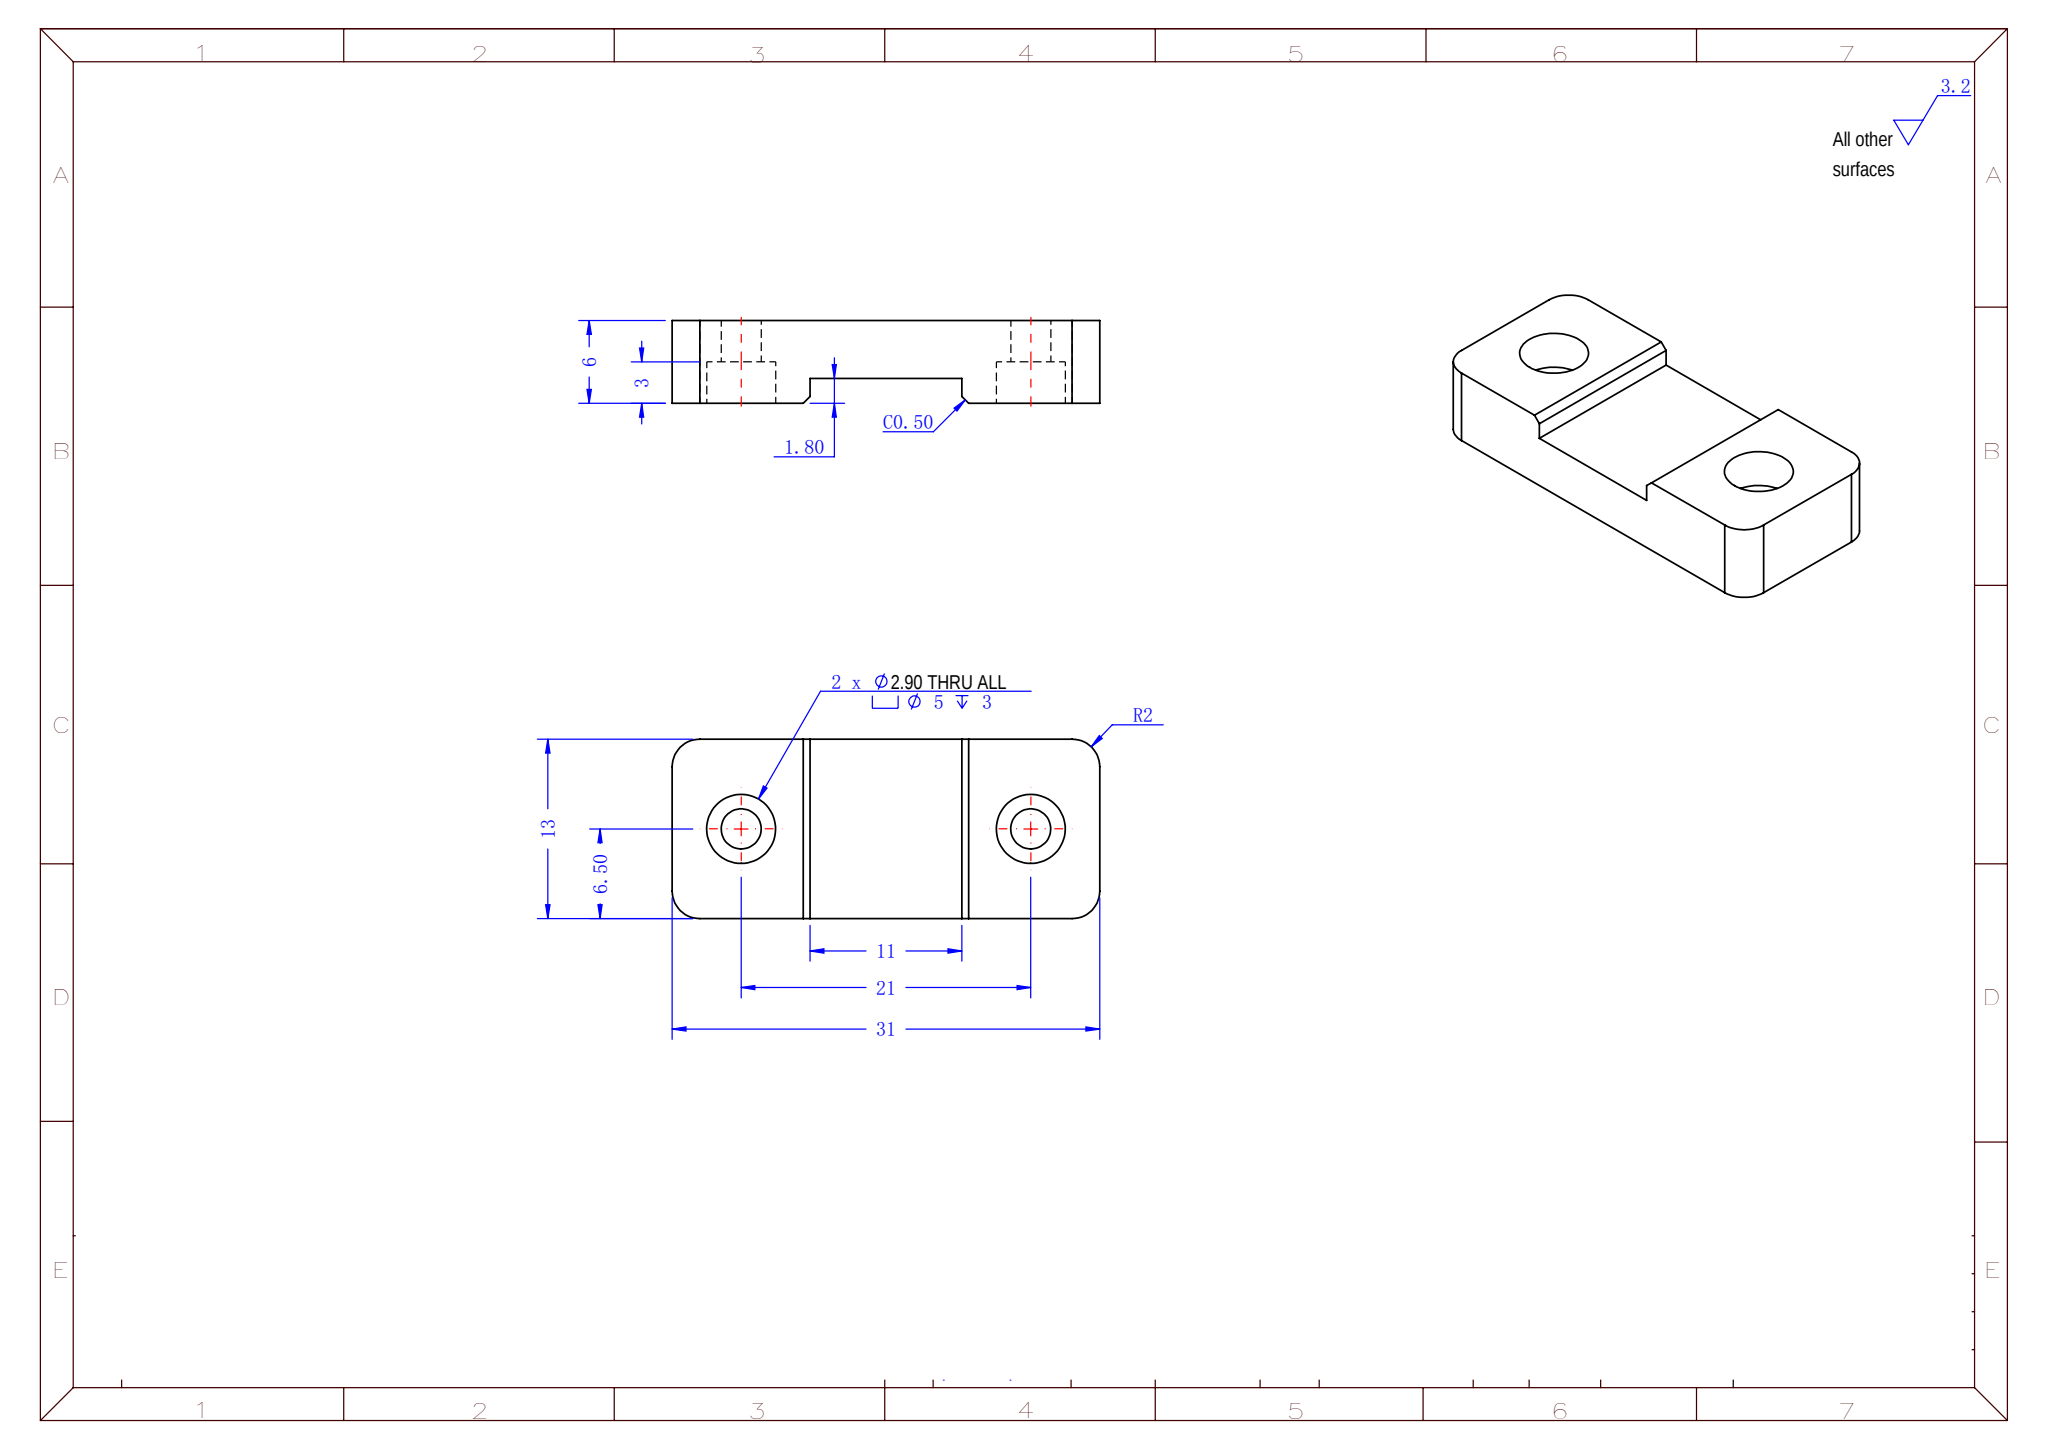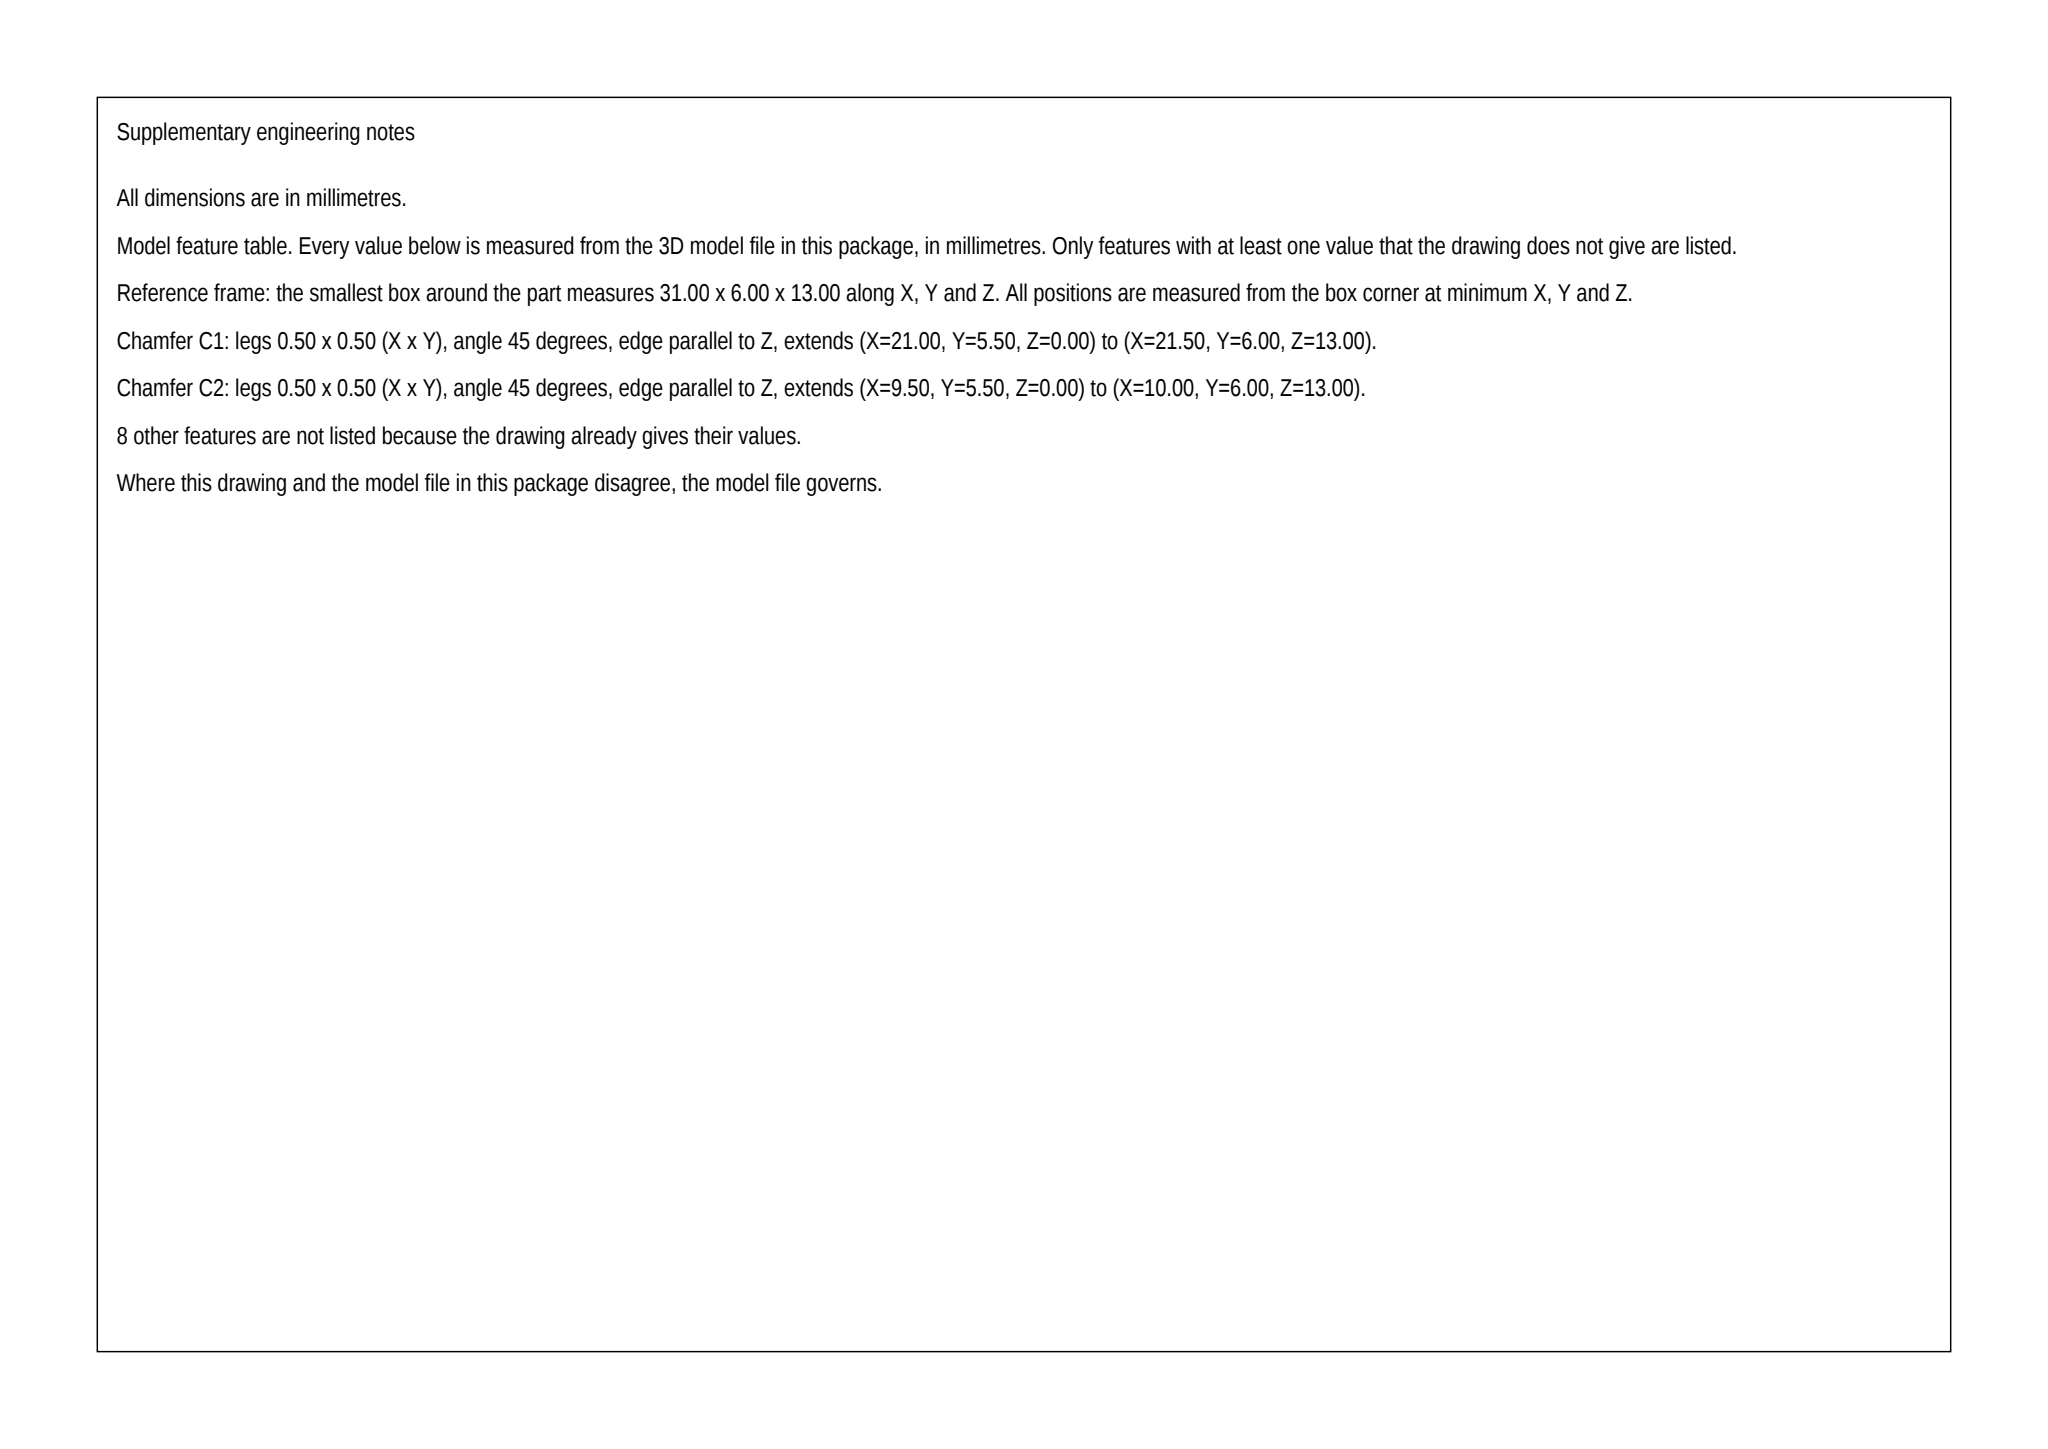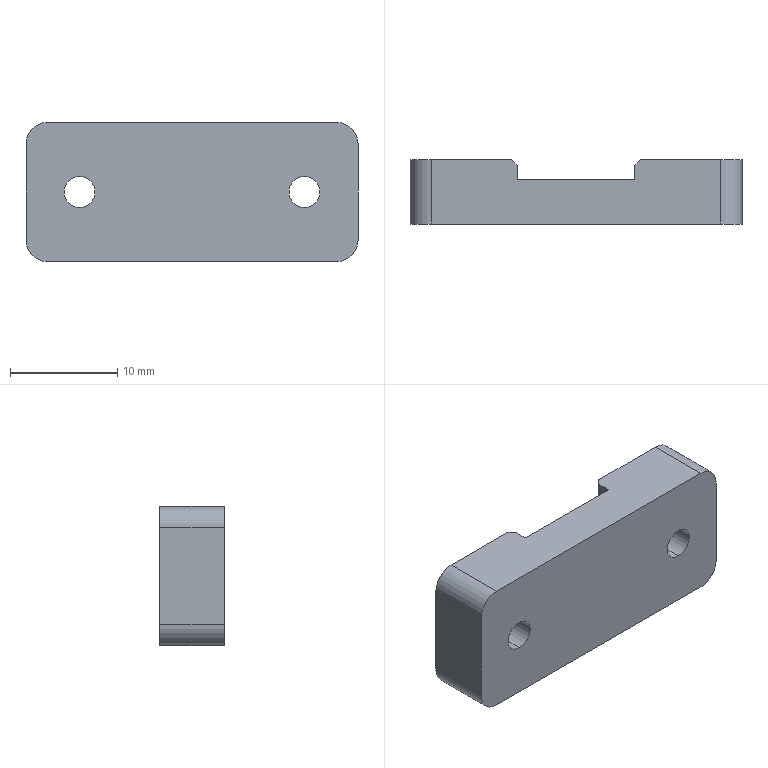Part | SolidWorks | mm | 1 solid | 26 faces | box 31 x 6 x 13 mm | volume 1979 mm3 | plane 14 | cylinder 12 | commonest cylinder face diameters 5 x4 2.9 x4 4 x4
build123d program:
from build123d import *

# Parameters (mm, degrees)
SKETCH1_W                                            = 31
SKETCH1_H                                            = 13
BOSS_EXTRUDE1_DEPTH                                  = 3
FILLET1_R                                            = 2
SKETCH3_W                                            = 11
SKETCH3_H                                            = 1.8
CUT_EXTRUDE2_DEPTH                                   = 21.451
CYLINDRICAL_COUNTERSUNK_HOLE_FOR_M2_5_HE_D           = 2.9
CYLINDRICAL_COUNTERSUNK_HOLE_FOR_M2_5_HE_CBORE_D     = 5
CYLINDRICAL_COUNTERSUNK_HOLE_FOR_M2_5_HE_CBORE_DEPTH = 3
CHAMFER1_SIZE                                        = 0.5


with BuildPart() as part:
    # Sketch1 → Boss-Extrude1 (new, symmetric)
    with BuildSketch(Plane(origin=(0, 0, 0), x_dir=(1, 0, 0), z_dir=(0, 1, 0))):
        Rectangle(SKETCH1_W, SKETCH1_H)
    extrude(amount=BOSS_EXTRUDE1_DEPTH, both=True)

    # Fillet1
    fillet1_edges = [part.edges().sort_by_distance(p)[0] for p in [
        (15.5, 0, 6.5),
        (-15.5, 0, 6.5),
        (-15.5, 0, -6.5),
        (15.5, 0, -6.5),
    ]]
    fillet(fillet1_edges, radius=FILLET1_R)

    # Sketch3 → Cut-Extrude2 (cut, through all)
    with BuildSketch(Plane(origin=(0, 0, -6.5), x_dir=(-1, 0, 0), z_dir=(0, 0, -1))):
        with Locations((0, 2.1)):
            Rectangle(SKETCH3_W, SKETCH3_H)
    extrude(amount=-CUT_EXTRUDE2_DEPTH, mode=Mode.SUBTRACT)

    # Cylindrical Countersunk Hole for M2.5 He (through all)
    with Locations(Plane(origin=(0, 3, 0), x_dir=(1, 0, 0), z_dir=(0, 1, 0))):
        with Locations((10.5, 0), (-10.5, 0)):
            CounterBoreHole(CYLINDRICAL_COUNTERSUNK_HOLE_FOR_M2_5_HE_D / 2, CYLINDRICAL_COUNTERSUNK_HOLE_FOR_M2_5_HE_CBORE_D / 2, CYLINDRICAL_COUNTERSUNK_HOLE_FOR_M2_5_HE_CBORE_DEPTH)

    # Chamfer1
    chamfer1_edges = [part.edges().sort_by_distance(p)[0] for p in [
        (5.5, 3, 0),
        (-5.5, 3, 0),
    ]]
    chamfer(chamfer1_edges, length=CHAMFER1_SIZE)


solid = part.part
STEP:
#1=CARTESIAN_POINT('',(10.5,0.,-2.5));
#2=VERTEX_POINT('',#1);
#3=CARTESIAN_POINT('',(10.5,0.,2.5));
#4=VERTEX_POINT('',#3);
#5=CARTESIAN_POINT('',(10.5,0.,0.));
#6=DIRECTION('',(0.,1.,0.));
#7=DIRECTION('',(0.,0.,1.));
#8=AXIS2_PLACEMENT_3D('',#5,#6,#7);
#9=CIRCLE('',#8,2.5);
#10=EDGE_CURVE('',#2,#4,#9,.T.);
#11=ORIENTED_EDGE('',*,*,#10,.F.);
#12=CARTESIAN_POINT('',(10.5,3.,-2.5));
#13=VERTEX_POINT('',#12);
#14=CARTESIAN_POINT('',(10.5,3.,-2.5));
#15=DIRECTION('',(0.,1.,0.));
#16=VECTOR('',#15,1000.);
#17=LINE('',#14,#16);
#18=EDGE_CURVE('',#2,#13,#17,.T.);
#19=ORIENTED_EDGE('',*,*,#18,.T.);
#20=CARTESIAN_POINT('',(10.5,3.,2.5));
#21=VERTEX_POINT('',#20);
#22=CARTESIAN_POINT('',(10.5,3.,0.));
#23=DIRECTION('',(0.,1.,0.));
#24=DIRECTION('',(0.,0.,1.));
#25=AXIS2_PLACEMENT_3D('',#22,#23,#24);
#26=CIRCLE('',#25,2.5);
#27=EDGE_CURVE('',#13,#21,#26,.T.);
#28=ORIENTED_EDGE('',*,*,#27,.T.);
#29=CARTESIAN_POINT('',(10.5,3.,2.5));
#30=DIRECTION('',(0.,1.,0.));
#31=VECTOR('',#30,1000.);
#32=LINE('',#29,#31);
#33=EDGE_CURVE('',#4,#21,#32,.T.);
#34=ORIENTED_EDGE('',*,*,#33,.F.);
#35=EDGE_LOOP('',(#11,#19,#28,#34));
#36=FACE_OUTER_BOUND('',#35,.T.);
#37=CARTESIAN_POINT('',(10.5,3.,0.));
#38=DIRECTION('',(0.,1.,0.));
#39=DIRECTION('',(0.,0.,1.));
#40=AXIS2_PLACEMENT_3D('',#37,#38,#39);
#41=CYLINDRICAL_SURFACE('',#40,2.5);
#42=ADVANCED_FACE('',(#36),#41,.F.);
#43=CARTESIAN_POINT('',(10.5,-3.,-1.45));
#44=VERTEX_POINT('',#43);
#45=CARTESIAN_POINT('',(10.5,-3.,1.45));
#46=VERTEX_POINT('',#45);
#47=CARTESIAN_POINT('',(10.5,-3.,0.));
#48=DIRECTION('',(0.,1.,0.));
#49=DIRECTION('',(0.,0.,1.));
#50=AXIS2_PLACEMENT_3D('',#47,#48,#49);
#51=CIRCLE('',#50,1.45);
#52=EDGE_CURVE('',#44,#46,#51,.T.);
#53=ORIENTED_EDGE('',*,*,#52,.F.);
#54=CARTESIAN_POINT('',(10.5,0.,-1.45));
#55=VERTEX_POINT('',#54);
#56=CARTESIAN_POINT('',(10.5,3.,-1.45));
#57=DIRECTION('',(0.,1.,0.));
#58=VECTOR('',#57,1000.);
#59=LINE('',#56,#58);
#60=EDGE_CURVE('',#44,#55,#59,.T.);
#61=ORIENTED_EDGE('',*,*,#60,.T.);
#62=CARTESIAN_POINT('',(10.5,0.,1.45));
#63=VERTEX_POINT('',#62);
#64=CARTESIAN_POINT('',(10.5,0.,0.));
#65=DIRECTION('',(0.,1.,0.));
#66=DIRECTION('',(0.,0.,1.));
#67=AXIS2_PLACEMENT_3D('',#64,#65,#66);
#68=CIRCLE('',#67,1.45);
#69=EDGE_CURVE('',#55,#63,#68,.T.);
#70=ORIENTED_EDGE('',*,*,#69,.T.);
#71=CARTESIAN_POINT('',(10.5,3.,1.45));
#72=DIRECTION('',(0.,1.,0.));
#73=VECTOR('',#72,1000.);
#74=LINE('',#71,#73);
#75=EDGE_CURVE('',#46,#63,#74,.T.);
#76=ORIENTED_EDGE('',*,*,#75,.F.);
#77=EDGE_LOOP('',(#53,#61,#70,#76));
#78=FACE_OUTER_BOUND('',#77,.T.);
#79=CARTESIAN_POINT('',(10.5,3.,0.));
#80=DIRECTION('',(0.,1.,0.));
#81=DIRECTION('',(0.,0.,1.));
#82=AXIS2_PLACEMENT_3D('',#79,#80,#81);
#83=CYLINDRICAL_SURFACE('',#82,1.45);
#84=ADVANCED_FACE('',(#78),#83,.F.);
#85=CARTESIAN_POINT('',(-10.5,0.,-2.5));
#86=VERTEX_POINT('',#85);
#87=CARTESIAN_POINT('',(-10.5,0.,2.5));
#88=VERTEX_POINT('',#87);
#89=CARTESIAN_POINT('',(-10.5,0.,0.));
#90=DIRECTION('',(0.,1.,0.));
#91=DIRECTION('',(0.,0.,1.));
#92=AXIS2_PLACEMENT_3D('',#89,#90,#91);
#93=CIRCLE('',#92,2.5);
#94=EDGE_CURVE('',#86,#88,#93,.T.);
#95=ORIENTED_EDGE('',*,*,#94,.F.);
#96=CARTESIAN_POINT('',(-10.5,3.,-2.5));
#97=VERTEX_POINT('',#96);
#98=CARTESIAN_POINT('',(-10.5,3.,-2.5));
#99=DIRECTION('',(0.,1.,0.));
#100=VECTOR('',#99,1000.);
#101=LINE('',#98,#100);
#102=EDGE_CURVE('',#86,#97,#101,.T.);
#103=ORIENTED_EDGE('',*,*,#102,.T.);
#104=CARTESIAN_POINT('',(-10.5,3.,2.5));
#105=VERTEX_POINT('',#104);
#106=CARTESIAN_POINT('',(-10.5,3.,0.));
#107=DIRECTION('',(0.,1.,0.));
#108=DIRECTION('',(0.,0.,1.));
#109=AXIS2_PLACEMENT_3D('',#106,#107,#108);
#110=CIRCLE('',#109,2.5);
#111=EDGE_CURVE('',#97,#105,#110,.T.);
#112=ORIENTED_EDGE('',*,*,#111,.T.);
#113=CARTESIAN_POINT('',(-10.5,3.,2.5));
#114=DIRECTION('',(0.,1.,0.));
#115=VECTOR('',#114,1000.);
#116=LINE('',#113,#115);
#117=EDGE_CURVE('',#88,#105,#116,.T.);
#118=ORIENTED_EDGE('',*,*,#117,.F.);
#119=EDGE_LOOP('',(#95,#103,#112,#118));
#120=FACE_OUTER_BOUND('',#119,.T.);
#121=CARTESIAN_POINT('',(-10.5,3.,0.));
#122=DIRECTION('',(0.,1.,0.));
#123=DIRECTION('',(0.,0.,1.));
#124=AXIS2_PLACEMENT_3D('',#121,#122,#123);
#125=CYLINDRICAL_SURFACE('',#124,2.5);
#126=ADVANCED_FACE('',(#120),#125,.F.);
#127=CARTESIAN_POINT('',(-10.5,-3.,-1.45));
#128=VERTEX_POINT('',#127);
#129=CARTESIAN_POINT('',(-10.5,-3.,1.45));
#130=VERTEX_POINT('',#129);
#131=CARTESIAN_POINT('',(-10.5,-3.,0.));
#132=DIRECTION('',(0.,1.,0.));
#133=DIRECTION('',(0.,0.,1.));
#134=AXIS2_PLACEMENT_3D('',#131,#132,#133);
#135=CIRCLE('',#134,1.45);
#136=EDGE_CURVE('',#128,#130,#135,.T.);
#137=ORIENTED_EDGE('',*,*,#136,.F.);
#138=CARTESIAN_POINT('',(-10.5,0.,-1.45));
#139=VERTEX_POINT('',#138);
#140=CARTESIAN_POINT('',(-10.5,3.,-1.45));
#141=DIRECTION('',(0.,1.,0.));
#142=VECTOR('',#141,1000.);
#143=LINE('',#140,#142);
#144=EDGE_CURVE('',#128,#139,#143,.T.);
#145=ORIENTED_EDGE('',*,*,#144,.T.);
#146=CARTESIAN_POINT('',(-10.5,0.,1.45));
#147=VERTEX_POINT('',#146);
#148=CARTESIAN_POINT('',(-10.5,0.,0.));
#149=DIRECTION('',(0.,1.,0.));
#150=DIRECTION('',(0.,0.,1.));
#151=AXIS2_PLACEMENT_3D('',#148,#149,#150);
#152=CIRCLE('',#151,1.45);
#153=EDGE_CURVE('',#139,#147,#152,.T.);
#154=ORIENTED_EDGE('',*,*,#153,.T.);
#155=CARTESIAN_POINT('',(-10.5,3.,1.45));
#156=DIRECTION('',(0.,1.,0.));
#157=VECTOR('',#156,1000.);
#158=LINE('',#155,#157);
#159=EDGE_CURVE('',#130,#147,#158,.T.);
#160=ORIENTED_EDGE('',*,*,#159,.F.);
#161=EDGE_LOOP('',(#137,#145,#154,#160));
#162=FACE_OUTER_BOUND('',#161,.T.);
#163=CARTESIAN_POINT('',(-10.5,3.,0.));
#164=DIRECTION('',(0.,1.,0.));
#165=DIRECTION('',(0.,0.,1.));
#166=AXIS2_PLACEMENT_3D('',#163,#164,#165);
#167=CYLINDRICAL_SURFACE('',#166,1.45);
#168=ADVANCED_FACE('',(#162),#167,.F.);
#169=CARTESIAN_POINT('',(-10.5,3.,0.));
#170=DIRECTION('',(0.,1.,0.));
#171=DIRECTION('',(0.,0.,1.));
#172=AXIS2_PLACEMENT_3D('',#169,#170,#171);
#173=CIRCLE('',#172,2.5);
#174=EDGE_CURVE('',#105,#97,#173,.T.);
#175=ORIENTED_EDGE('',*,*,#174,.F.);
#176=ORIENTED_EDGE('',*,*,#111,.F.);
#177=EDGE_LOOP('',(#175,#176));
#178=FACE_BOUND('',#177,.T.);
#179=CARTESIAN_POINT('',(-13.5,3.,6.5));
#180=VERTEX_POINT('',#179);
#181=CARTESIAN_POINT('',(-6.,3.,6.5));
#182=VERTEX_POINT('',#181);
#183=CARTESIAN_POINT('',(-15.5,3.,6.5));
#184=DIRECTION('',(1.,0.,0.));
#185=VECTOR('',#184,1000.);
#186=LINE('',#183,#185);
#187=EDGE_CURVE('',#180,#182,#186,.T.);
#188=ORIENTED_EDGE('',*,*,#187,.T.);
#189=CARTESIAN_POINT('',(-6.,3.,-6.5));
#190=VERTEX_POINT('',#189);
#191=CARTESIAN_POINT('',(-6.,3.,-6.5));
#192=DIRECTION('',(0.,0.,-1.));
#193=VECTOR('',#192,1000.);
#194=LINE('',#191,#193);
#195=EDGE_CURVE('',#182,#190,#194,.T.);
#196=ORIENTED_EDGE('',*,*,#195,.T.);
#197=CARTESIAN_POINT('',(-13.5,3.,-6.5));
#198=VERTEX_POINT('',#197);
#199=CARTESIAN_POINT('',(-15.5,3.,-6.5));
#200=DIRECTION('',(-1.,0.,0.));
#201=VECTOR('',#200,1000.);
#202=LINE('',#199,#201);
#203=EDGE_CURVE('',#190,#198,#202,.T.);
#204=ORIENTED_EDGE('',*,*,#203,.T.);
#205=CARTESIAN_POINT('',(-15.5,3.,-4.5));
#206=VERTEX_POINT('',#205);
#207=CARTESIAN_POINT('',(-13.5,3.,-4.5));
#208=DIRECTION('',(0.,1.,0.));
#209=DIRECTION('',(0.,0.,1.));
#210=AXIS2_PLACEMENT_3D('',#207,#208,#209);
#211=CIRCLE('',#210,2.);
#212=EDGE_CURVE('',#198,#206,#211,.T.);
#213=ORIENTED_EDGE('',*,*,#212,.T.);
#214=CARTESIAN_POINT('',(-15.5,3.,4.5));
#215=VERTEX_POINT('',#214);
#216=CARTESIAN_POINT('',(-15.5,3.,-6.5));
#217=DIRECTION('',(0.,0.,1.));
#218=VECTOR('',#217,1000.);
#219=LINE('',#216,#218);
#220=EDGE_CURVE('',#206,#215,#219,.T.);
#221=ORIENTED_EDGE('',*,*,#220,.T.);
#222=CARTESIAN_POINT('',(-13.5,3.,4.5));
#223=DIRECTION('',(0.,1.,0.));
#224=DIRECTION('',(0.,0.,1.));
#225=AXIS2_PLACEMENT_3D('',#222,#223,#224);
#226=CIRCLE('',#225,2.);
#227=EDGE_CURVE('',#215,#180,#226,.T.);
#228=ORIENTED_EDGE('',*,*,#227,.T.);
#229=EDGE_LOOP('',(#188,#196,#204,#213,#221,#228));
#230=FACE_OUTER_BOUND('',#229,.T.);
#231=CARTESIAN_POINT('',(0.,3.,0.));
#232=DIRECTION('',(0.,1.,0.));
#233=DIRECTION('',(0.,0.,1.));
#234=AXIS2_PLACEMENT_3D('',#231,#232,#233);
#235=PLANE('',#234);
#236=ADVANCED_FACE('',(#178,#230),#235,.T.);
#237=CARTESIAN_POINT('',(15.5,3.,4.5));
#238=VERTEX_POINT('',#237);
#239=CARTESIAN_POINT('',(15.5,3.,-4.5));
#240=VERTEX_POINT('',#239);
#241=CARTESIAN_POINT('',(15.5,3.,-6.5));
#242=DIRECTION('',(-0.,0.,-1.));
#243=VECTOR('',#242,1000.);
#244=LINE('',#241,#243);
#245=EDGE_CURVE('',#238,#240,#244,.T.);
#246=ORIENTED_EDGE('',*,*,#245,.F.);
#247=CARTESIAN_POINT('',(15.5,-3.,4.5));
#248=VERTEX_POINT('',#247);
#249=CARTESIAN_POINT('',(15.5,3.,4.5));
#250=DIRECTION('',(0.,-1.,0.));
#251=VECTOR('',#250,1000.);
#252=LINE('',#249,#251);
#253=EDGE_CURVE('',#238,#248,#252,.T.);
#254=ORIENTED_EDGE('',*,*,#253,.T.);
#255=CARTESIAN_POINT('',(15.5,-3.,-4.5));
#256=VERTEX_POINT('',#255);
#257=CARTESIAN_POINT('',(15.5,-3.,-6.5));
#258=DIRECTION('',(-0.,0.,-1.));
#259=VECTOR('',#258,1000.);
#260=LINE('',#257,#259);
#261=EDGE_CURVE('',#248,#256,#260,.T.);
#262=ORIENTED_EDGE('',*,*,#261,.T.);
#263=CARTESIAN_POINT('',(15.5,3.,-4.5));
#264=DIRECTION('',(0.,1.,0.));
#265=VECTOR('',#264,1000.);
#266=LINE('',#263,#265);
#267=EDGE_CURVE('',#256,#240,#266,.T.);
#268=ORIENTED_EDGE('',*,*,#267,.T.);
#269=EDGE_LOOP('',(#246,#254,#262,#268));
#270=FACE_OUTER_BOUND('',#269,.T.);
#271=CARTESIAN_POINT('',(15.5,3.,-6.5));
#272=DIRECTION('',(-1.,0.,0.));
#273=DIRECTION('',(0.,0.,1.));
#274=AXIS2_PLACEMENT_3D('',#271,#272,#273);
#275=PLANE('',#274);
#276=ADVANCED_FACE('',(#270),#275,.F.);
#277=CARTESIAN_POINT('',(5.5,2.5,-6.5));
#278=VERTEX_POINT('',#277);
#279=CARTESIAN_POINT('',(5.5,1.2,-6.5));
#280=VERTEX_POINT('',#279);
#281=CARTESIAN_POINT('',(5.5,3.,-6.5));
#282=DIRECTION('',(0.,-1.,0.));
#283=VECTOR('',#282,1000.);
#284=LINE('',#281,#283);
#285=EDGE_CURVE('',#278,#280,#284,.T.);
#286=ORIENTED_EDGE('',*,*,#285,.F.);
#287=CARTESIAN_POINT('',(6.,3.,-6.5));
#288=VERTEX_POINT('',#287);
#289=CARTESIAN_POINT('',(5.5,2.5,-6.5));
#290=DIRECTION('',(0.7071,0.7071,0.));
#291=VECTOR('',#290,1000.);
#292=LINE('',#289,#291);
#293=EDGE_CURVE('',#278,#288,#292,.T.);
#294=ORIENTED_EDGE('',*,*,#293,.T.);
#295=CARTESIAN_POINT('',(13.5,3.,-6.5));
#296=VERTEX_POINT('',#295);
#297=CARTESIAN_POINT('',(-15.5,3.,-6.5));
#298=DIRECTION('',(-1.,0.,0.));
#299=VECTOR('',#298,1000.);
#300=LINE('',#297,#299);
#301=EDGE_CURVE('',#296,#288,#300,.T.);
#302=ORIENTED_EDGE('',*,*,#301,.F.);
#303=CARTESIAN_POINT('',(13.5,-3.,-6.5));
#304=VERTEX_POINT('',#303);
#305=CARTESIAN_POINT('',(13.5,3.,-6.5));
#306=DIRECTION('',(0.,-1.,0.));
#307=VECTOR('',#306,1000.);
#308=LINE('',#305,#307);
#309=EDGE_CURVE('',#296,#304,#308,.T.);
#310=ORIENTED_EDGE('',*,*,#309,.T.);
#311=CARTESIAN_POINT('',(-13.5,-3.,-6.5));
#312=VERTEX_POINT('',#311);
#313=CARTESIAN_POINT('',(-15.5,-3.,-6.5));
#314=DIRECTION('',(-1.,0.,0.));
#315=VECTOR('',#314,1000.);
#316=LINE('',#313,#315);
#317=EDGE_CURVE('',#304,#312,#316,.T.);
#318=ORIENTED_EDGE('',*,*,#317,.T.);
#319=CARTESIAN_POINT('',(-13.5,3.,-6.5));
#320=DIRECTION('',(0.,1.,0.));
#321=VECTOR('',#320,1000.);
#322=LINE('',#319,#321);
#323=EDGE_CURVE('',#312,#198,#322,.T.);
#324=ORIENTED_EDGE('',*,*,#323,.T.);
#325=ORIENTED_EDGE('',*,*,#203,.F.);
#326=CARTESIAN_POINT('',(-5.5,2.5,-6.5));
#327=VERTEX_POINT('',#326);
#328=CARTESIAN_POINT('',(-6.,3.,-6.5));
#329=DIRECTION('',(0.7071,-0.7071,0.));
#330=VECTOR('',#329,1000.);
#331=LINE('',#328,#330);
#332=EDGE_CURVE('',#190,#327,#331,.T.);
#333=ORIENTED_EDGE('',*,*,#332,.T.);
#334=CARTESIAN_POINT('',(-5.5,1.2,-6.5));
#335=VERTEX_POINT('',#334);
#336=CARTESIAN_POINT('',(-5.5,1.2,-6.5));
#337=DIRECTION('',(0.,1.,0.));
#338=VECTOR('',#337,1000.);
#339=LINE('',#336,#338);
#340=EDGE_CURVE('',#335,#327,#339,.T.);
#341=ORIENTED_EDGE('',*,*,#340,.F.);
#342=CARTESIAN_POINT('',(5.5,1.2,-6.5));
#343=DIRECTION('',(-1.,0.,0.));
#344=VECTOR('',#343,1000.);
#345=LINE('',#342,#344);
#346=EDGE_CURVE('',#280,#335,#345,.T.);
#347=ORIENTED_EDGE('',*,*,#346,.F.);
#348=EDGE_LOOP('',(#286,#294,#302,#310,#318,#324,#325,#333,#341,#347));
#349=FACE_OUTER_BOUND('',#348,.T.);
#350=CARTESIAN_POINT('',(-15.5,3.,-6.5));
#351=DIRECTION('',(0.,0.,1.));
#352=DIRECTION('',(1.,0.,0.));
#353=AXIS2_PLACEMENT_3D('',#350,#351,#352);
#354=PLANE('',#353);
#355=ADVANCED_FACE('',(#349),#354,.F.);
#356=ORIENTED_EDGE('',*,*,#220,.F.);
#357=CARTESIAN_POINT('',(-15.5,-3.,-4.5));
#358=VERTEX_POINT('',#357);
#359=CARTESIAN_POINT('',(-15.5,3.,-4.5));
#360=DIRECTION('',(0.,-1.,0.));
#361=VECTOR('',#360,1000.);
#362=LINE('',#359,#361);
#363=EDGE_CURVE('',#206,#358,#362,.T.);
#364=ORIENTED_EDGE('',*,*,#363,.T.);
#365=CARTESIAN_POINT('',(-15.5,-3.,4.5));
#366=VERTEX_POINT('',#365);
#367=CARTESIAN_POINT('',(-15.5,-3.,-6.5));
#368=DIRECTION('',(0.,0.,1.));
#369=VECTOR('',#368,1000.);
#370=LINE('',#367,#369);
#371=EDGE_CURVE('',#358,#366,#370,.T.);
#372=ORIENTED_EDGE('',*,*,#371,.T.);
#373=CARTESIAN_POINT('',(-15.5,3.,4.5));
#374=DIRECTION('',(0.,1.,0.));
#375=VECTOR('',#374,1000.);
#376=LINE('',#373,#375);
#377=EDGE_CURVE('',#366,#215,#376,.T.);
#378=ORIENTED_EDGE('',*,*,#377,.T.);
#379=EDGE_LOOP('',(#356,#364,#372,#378));
#380=FACE_OUTER_BOUND('',#379,.T.);
#381=CARTESIAN_POINT('',(-15.5,3.,-6.5));
#382=DIRECTION('',(1.,0.,-0.));
#383=DIRECTION('',(-0.,0.,-1.));
#384=AXIS2_PLACEMENT_3D('',#381,#382,#383);
#385=PLANE('',#384);
#386=ADVANCED_FACE('',(#380),#385,.F.);
#387=CARTESIAN_POINT('',(6.,3.,6.5));
#388=VERTEX_POINT('',#387);
#389=CARTESIAN_POINT('',(13.5,3.,6.5));
#390=VERTEX_POINT('',#389);
#391=CARTESIAN_POINT('',(-15.5,3.,6.5));
#392=DIRECTION('',(1.,0.,0.));
#393=VECTOR('',#392,1000.);
#394=LINE('',#391,#393);
#395=EDGE_CURVE('',#388,#390,#394,.T.);
#396=ORIENTED_EDGE('',*,*,#395,.F.);
#397=CARTESIAN_POINT('',(5.5,2.5,6.5));
#398=VERTEX_POINT('',#397);
#399=CARTESIAN_POINT('',(5.5,2.5,6.5));
#400=DIRECTION('',(-0.7071,-0.7071,0.));
#401=VECTOR('',#400,1000.);
#402=LINE('',#399,#401);
#403=EDGE_CURVE('',#388,#398,#402,.T.);
#404=ORIENTED_EDGE('',*,*,#403,.T.);
#405=CARTESIAN_POINT('',(5.5,1.2,6.5));
#406=VERTEX_POINT('',#405);
#407=CARTESIAN_POINT('',(5.5,3.,6.5));
#408=DIRECTION('',(0.,-1.,0.));
#409=VECTOR('',#408,1000.);
#410=LINE('',#407,#409);
#411=EDGE_CURVE('',#398,#406,#410,.T.);
#412=ORIENTED_EDGE('',*,*,#411,.T.);
#413=CARTESIAN_POINT('',(-5.5,1.2,6.5));
#414=VERTEX_POINT('',#413);
#415=CARTESIAN_POINT('',(5.5,1.2,6.5));
#416=DIRECTION('',(-1.,0.,0.));
#417=VECTOR('',#416,1000.);
#418=LINE('',#415,#417);
#419=EDGE_CURVE('',#406,#414,#418,.T.);
#420=ORIENTED_EDGE('',*,*,#419,.T.);
#421=CARTESIAN_POINT('',(-5.5,2.5,6.5));
#422=VERTEX_POINT('',#421);
#423=CARTESIAN_POINT('',(-5.5,1.2,6.5));
#424=DIRECTION('',(0.,1.,0.));
#425=VECTOR('',#424,1000.);
#426=LINE('',#423,#425);
#427=EDGE_CURVE('',#414,#422,#426,.T.);
#428=ORIENTED_EDGE('',*,*,#427,.T.);
#429=CARTESIAN_POINT('',(-6.,3.,6.5));
#430=DIRECTION('',(-0.7071,0.7071,0.));
#431=VECTOR('',#430,1000.);
#432=LINE('',#429,#431);
#433=EDGE_CURVE('',#422,#182,#432,.T.);
#434=ORIENTED_EDGE('',*,*,#433,.T.);
#435=ORIENTED_EDGE('',*,*,#187,.F.);
#436=CARTESIAN_POINT('',(-13.5,-3.,6.5));
#437=VERTEX_POINT('',#436);
#438=CARTESIAN_POINT('',(-13.5,3.,6.5));
#439=DIRECTION('',(0.,-1.,0.));
#440=VECTOR('',#439,1000.);
#441=LINE('',#438,#440);
#442=EDGE_CURVE('',#180,#437,#441,.T.);
#443=ORIENTED_EDGE('',*,*,#442,.T.);
#444=CARTESIAN_POINT('',(13.5,-3.,6.5));
#445=VERTEX_POINT('',#444);
#446=CARTESIAN_POINT('',(-15.5,-3.,6.5));
#447=DIRECTION('',(1.,0.,0.));
#448=VECTOR('',#447,1000.);
#449=LINE('',#446,#448);
#450=EDGE_CURVE('',#437,#445,#449,.T.);
#451=ORIENTED_EDGE('',*,*,#450,.T.);
#452=CARTESIAN_POINT('',(13.5,3.,6.5));
#453=DIRECTION('',(0.,1.,0.));
#454=VECTOR('',#453,1000.);
#455=LINE('',#452,#454);
#456=EDGE_CURVE('',#445,#390,#455,.T.);
#457=ORIENTED_EDGE('',*,*,#456,.T.);
#458=EDGE_LOOP('',(#396,#404,#412,#420,#428,#434,#435,#443,#451,#457));
#459=FACE_OUTER_BOUND('',#458,.T.);
#460=CARTESIAN_POINT('',(-15.5,3.,6.5));
#461=DIRECTION('',(0.,0.,-1.));
#462=DIRECTION('',(-1.,0.,0.));
#463=AXIS2_PLACEMENT_3D('',#460,#461,#462);
#464=PLANE('',#463);
#465=ADVANCED_FACE('',(#459),#464,.F.);
#466=CARTESIAN_POINT('',(10.5,3.,0.));
#467=DIRECTION('',(0.,1.,0.));
#468=DIRECTION('',(0.,0.,1.));
#469=AXIS2_PLACEMENT_3D('',#466,#467,#468);
#470=CIRCLE('',#469,2.5);
#471=EDGE_CURVE('',#21,#13,#470,.T.);
#472=ORIENTED_EDGE('',*,*,#471,.F.);
#473=ORIENTED_EDGE('',*,*,#27,.F.);
#474=EDGE_LOOP('',(#472,#473));
#475=FACE_BOUND('',#474,.T.);
#476=ORIENTED_EDGE('',*,*,#301,.T.);
#477=CARTESIAN_POINT('',(6.,3.,6.5));
#478=DIRECTION('',(0.,0.,1.));
#479=VECTOR('',#478,1000.);
#480=LINE('',#477,#479);
#481=EDGE_CURVE('',#288,#388,#480,.T.);
#482=ORIENTED_EDGE('',*,*,#481,.T.);
#483=ORIENTED_EDGE('',*,*,#395,.T.);
#484=CARTESIAN_POINT('',(13.5,3.,4.5));
#485=DIRECTION('',(0.,1.,0.));
#486=DIRECTION('',(0.,0.,1.));
#487=AXIS2_PLACEMENT_3D('',#484,#485,#486);
#488=CIRCLE('',#487,2.);
#489=EDGE_CURVE('',#390,#238,#488,.T.);
#490=ORIENTED_EDGE('',*,*,#489,.T.);
#491=ORIENTED_EDGE('',*,*,#245,.T.);
#492=CARTESIAN_POINT('',(13.5,3.,-4.5));
#493=DIRECTION('',(0.,1.,0.));
#494=DIRECTION('',(0.,0.,1.));
#495=AXIS2_PLACEMENT_3D('',#492,#493,#494);
#496=CIRCLE('',#495,2.);
#497=EDGE_CURVE('',#240,#296,#496,.T.);
#498=ORIENTED_EDGE('',*,*,#497,.T.);
#499=EDGE_LOOP('',(#476,#482,#483,#490,#491,#498));
#500=FACE_OUTER_BOUND('',#499,.T.);
#501=CARTESIAN_POINT('',(0.,3.,0.));
#502=DIRECTION('',(0.,1.,0.));
#503=DIRECTION('',(0.,0.,1.));
#504=AXIS2_PLACEMENT_3D('',#501,#502,#503);
#505=PLANE('',#504);
#506=ADVANCED_FACE('',(#475,#500),#505,.T.);
#507=CARTESIAN_POINT('',(10.5,-3.,0.));
#508=DIRECTION('',(0.,1.,0.));
#509=DIRECTION('',(0.,0.,1.));
#510=AXIS2_PLACEMENT_3D('',#507,#508,#509);
#511=CIRCLE('',#510,1.45);
#512=EDGE_CURVE('',#46,#44,#511,.T.);
#513=ORIENTED_EDGE('',*,*,#512,.T.);
#514=ORIENTED_EDGE('',*,*,#52,.T.);
#515=EDGE_LOOP('',(#513,#514));
#516=FACE_BOUND('',#515,.T.);
#517=CARTESIAN_POINT('',(-10.5,-3.,0.));
#518=DIRECTION('',(0.,1.,0.));
#519=DIRECTION('',(0.,0.,1.));
#520=AXIS2_PLACEMENT_3D('',#517,#518,#519);
#521=CIRCLE('',#520,1.45);
#522=EDGE_CURVE('',#130,#128,#521,.T.);
#523=ORIENTED_EDGE('',*,*,#522,.T.);
#524=ORIENTED_EDGE('',*,*,#136,.T.);
#525=EDGE_LOOP('',(#523,#524));
#526=FACE_BOUND('',#525,.T.);
#527=ORIENTED_EDGE('',*,*,#261,.F.);
#528=CARTESIAN_POINT('',(13.5,-3.,4.5));
#529=DIRECTION('',(0.,-1.,0.));
#530=DIRECTION('',(0.,0.,1.));
#531=AXIS2_PLACEMENT_3D('',#528,#529,#530);
#532=CIRCLE('',#531,2.);
#533=EDGE_CURVE('',#248,#445,#532,.T.);
#534=ORIENTED_EDGE('',*,*,#533,.T.);
#535=ORIENTED_EDGE('',*,*,#450,.F.);
#536=CARTESIAN_POINT('',(-13.5,-3.,4.5));
#537=DIRECTION('',(0.,-1.,0.));
#538=DIRECTION('',(0.,0.,1.));
#539=AXIS2_PLACEMENT_3D('',#536,#537,#538);
#540=CIRCLE('',#539,2.);
#541=EDGE_CURVE('',#437,#366,#540,.T.);
#542=ORIENTED_EDGE('',*,*,#541,.T.);
#543=ORIENTED_EDGE('',*,*,#371,.F.);
#544=CARTESIAN_POINT('',(-13.5,-3.,-4.5));
#545=DIRECTION('',(0.,-1.,0.));
#546=DIRECTION('',(0.,0.,1.));
#547=AXIS2_PLACEMENT_3D('',#544,#545,#546);
#548=CIRCLE('',#547,2.);
#549=EDGE_CURVE('',#358,#312,#548,.T.);
#550=ORIENTED_EDGE('',*,*,#549,.T.);
#551=ORIENTED_EDGE('',*,*,#317,.F.);
#552=CARTESIAN_POINT('',(13.5,-3.,-4.5));
#553=DIRECTION('',(0.,-1.,0.));
#554=DIRECTION('',(-0.,0.,1.));
#555=AXIS2_PLACEMENT_3D('',#552,#553,#554);
#556=CIRCLE('',#555,2.);
#557=EDGE_CURVE('',#304,#256,#556,.T.);
#558=ORIENTED_EDGE('',*,*,#557,.T.);
#559=EDGE_LOOP('',(#527,#534,#535,#542,#543,#550,#551,#558));
#560=FACE_OUTER_BOUND('',#559,.T.);
#561=CARTESIAN_POINT('',(0.,-3.,0.));
#562=DIRECTION('',(0.,1.,0.));
#563=DIRECTION('',(0.,0.,1.));
#564=AXIS2_PLACEMENT_3D('',#561,#562,#563);
#565=PLANE('',#564);
#566=ADVANCED_FACE('',(#516,#526,#560),#565,.F.);
#567=ORIENTED_EDGE('',*,*,#489,.F.);
#568=ORIENTED_EDGE('',*,*,#456,.F.);
#569=ORIENTED_EDGE('',*,*,#533,.F.);
#570=ORIENTED_EDGE('',*,*,#253,.F.);
#571=EDGE_LOOP('',(#567,#568,#569,#570));
#572=FACE_OUTER_BOUND('',#571,.T.);
#573=CARTESIAN_POINT('',(13.5,3.,4.5));
#574=DIRECTION('',(0.,-1.,0.));
#575=DIRECTION('',(0.,0.,-1.));
#576=AXIS2_PLACEMENT_3D('',#573,#574,#575);
#577=CYLINDRICAL_SURFACE('',#576,2.);
#578=ADVANCED_FACE('',(#572),#577,.T.);
#579=ORIENTED_EDGE('',*,*,#212,.F.);
#580=ORIENTED_EDGE('',*,*,#323,.F.);
#581=ORIENTED_EDGE('',*,*,#549,.F.);
#582=ORIENTED_EDGE('',*,*,#363,.F.);
#583=EDGE_LOOP('',(#579,#580,#581,#582));
#584=FACE_OUTER_BOUND('',#583,.T.);
#585=CARTESIAN_POINT('',(-13.5,3.,-4.5));
#586=DIRECTION('',(0.,-1.,0.));
#587=DIRECTION('',(0.,0.,-1.));
#588=AXIS2_PLACEMENT_3D('',#585,#586,#587);
#589=CYLINDRICAL_SURFACE('',#588,2.);
#590=ADVANCED_FACE('',(#584),#589,.T.);
#591=ORIENTED_EDGE('',*,*,#497,.F.);
#592=ORIENTED_EDGE('',*,*,#267,.F.);
#593=ORIENTED_EDGE('',*,*,#557,.F.);
#594=ORIENTED_EDGE('',*,*,#309,.F.);
#595=EDGE_LOOP('',(#591,#592,#593,#594));
#596=FACE_OUTER_BOUND('',#595,.T.);
#597=CARTESIAN_POINT('',(13.5,3.,-4.5));
#598=DIRECTION('',(0.,-1.,0.));
#599=DIRECTION('',(0.,0.,-1.));
#600=AXIS2_PLACEMENT_3D('',#597,#598,#599);
#601=CYLINDRICAL_SURFACE('',#600,2.);
#602=ADVANCED_FACE('',(#596),#601,.T.);
#603=ORIENTED_EDGE('',*,*,#227,.F.);
#604=ORIENTED_EDGE('',*,*,#377,.F.);
#605=ORIENTED_EDGE('',*,*,#541,.F.);
#606=ORIENTED_EDGE('',*,*,#442,.F.);
#607=EDGE_LOOP('',(#603,#604,#605,#606));
#608=FACE_OUTER_BOUND('',#607,.T.);
#609=CARTESIAN_POINT('',(-13.5,3.,4.5));
#610=DIRECTION('',(0.,-1.,0.));
#611=DIRECTION('',(0.,0.,-1.));
#612=AXIS2_PLACEMENT_3D('',#609,#610,#611);
#613=CYLINDRICAL_SURFACE('',#612,2.);
#614=ADVANCED_FACE('',(#608),#613,.T.);
#615=ORIENTED_EDGE('',*,*,#340,.T.);
#616=CARTESIAN_POINT('',(-5.5,2.5,6.5));
#617=DIRECTION('',(0.,0.,1.));
#618=VECTOR('',#617,1000.);
#619=LINE('',#616,#618);
#620=EDGE_CURVE('',#327,#422,#619,.T.);
#621=ORIENTED_EDGE('',*,*,#620,.T.);
#622=ORIENTED_EDGE('',*,*,#427,.F.);
#623=CARTESIAN_POINT('',(-5.5,1.2,6.5));
#624=DIRECTION('',(0.,0.,-1.));
#625=VECTOR('',#624,1000.);
#626=LINE('',#623,#625);
#627=EDGE_CURVE('',#414,#335,#626,.T.);
#628=ORIENTED_EDGE('',*,*,#627,.T.);
#629=EDGE_LOOP('',(#615,#621,#622,#628));
#630=FACE_OUTER_BOUND('',#629,.T.);
#631=CARTESIAN_POINT('',(-5.5,1.2,6.5));
#632=DIRECTION('',(-1.,0.,0.));
#633=DIRECTION('',(0.,0.,1.));
#634=AXIS2_PLACEMENT_3D('',#631,#632,#633);
#635=PLANE('',#634);
#636=ADVANCED_FACE('',(#630),#635,.F.);
#637=ORIENTED_EDGE('',*,*,#346,.T.);
#638=ORIENTED_EDGE('',*,*,#627,.F.);
#639=ORIENTED_EDGE('',*,*,#419,.F.);
#640=CARTESIAN_POINT('',(5.5,1.2,6.5));
#641=DIRECTION('',(0.,0.,-1.));
#642=VECTOR('',#641,1000.);
#643=LINE('',#640,#642);
#644=EDGE_CURVE('',#406,#280,#643,.T.);
#645=ORIENTED_EDGE('',*,*,#644,.T.);
#646=EDGE_LOOP('',(#637,#638,#639,#645));
#647=FACE_OUTER_BOUND('',#646,.T.);
#648=CARTESIAN_POINT('',(5.5,1.2,6.5));
#649=DIRECTION('',(-0.,-1.,0.));
#650=DIRECTION('',(1.,-0.,0.));
#651=AXIS2_PLACEMENT_3D('',#648,#649,#650);
#652=PLANE('',#651);
#653=ADVANCED_FACE('',(#647),#652,.F.);
#654=ORIENTED_EDGE('',*,*,#411,.F.);
#655=CARTESIAN_POINT('',(5.5,2.5,-6.5));
#656=DIRECTION('',(0.,0.,-1.));
#657=VECTOR('',#656,1000.);
#658=LINE('',#655,#657);
#659=EDGE_CURVE('',#398,#278,#658,.T.);
#660=ORIENTED_EDGE('',*,*,#659,.T.);
#661=ORIENTED_EDGE('',*,*,#285,.T.);
#662=ORIENTED_EDGE('',*,*,#644,.F.);
#663=EDGE_LOOP('',(#654,#660,#661,#662));
#664=FACE_OUTER_BOUND('',#663,.T.);
#665=CARTESIAN_POINT('',(5.5,3.,6.5));
#666=DIRECTION('',(1.,0.,0.));
#667=DIRECTION('',(0.,0.,-1.));
#668=AXIS2_PLACEMENT_3D('',#665,#666,#667);
#669=PLANE('',#668);
#670=ADVANCED_FACE('',(#664),#669,.F.);
#671=ORIENTED_EDGE('',*,*,#144,.F.);
#672=ORIENTED_EDGE('',*,*,#522,.F.);
#673=ORIENTED_EDGE('',*,*,#159,.T.);
#674=CARTESIAN_POINT('',(-10.5,0.,0.));
#675=DIRECTION('',(0.,1.,0.));
#676=DIRECTION('',(0.,0.,1.));
#677=AXIS2_PLACEMENT_3D('',#674,#675,#676);
#678=CIRCLE('',#677,1.45);
#679=EDGE_CURVE('',#147,#139,#678,.T.);
#680=ORIENTED_EDGE('',*,*,#679,.T.);
#681=EDGE_LOOP('',(#671,#672,#673,#680));
#682=FACE_OUTER_BOUND('',#681,.T.);
#683=CARTESIAN_POINT('',(-10.5,3.,0.));
#684=DIRECTION('',(0.,1.,0.));
#685=DIRECTION('',(0.,0.,1.));
#686=AXIS2_PLACEMENT_3D('',#683,#684,#685);
#687=CYLINDRICAL_SURFACE('',#686,1.45);
#688=ADVANCED_FACE('',(#682),#687,.F.);
#689=ORIENTED_EDGE('',*,*,#679,.F.);
#690=ORIENTED_EDGE('',*,*,#153,.F.);
#691=EDGE_LOOP('',(#689,#690));
#692=FACE_BOUND('',#691,.T.);
#693=CARTESIAN_POINT('',(-10.5,0.,0.));
#694=DIRECTION('',(0.,1.,0.));
#695=DIRECTION('',(0.,0.,1.));
#696=AXIS2_PLACEMENT_3D('',#693,#694,#695);
#697=CIRCLE('',#696,2.5);
#698=EDGE_CURVE('',#88,#86,#697,.T.);
#699=ORIENTED_EDGE('',*,*,#698,.T.);
#700=ORIENTED_EDGE('',*,*,#94,.T.);
#701=EDGE_LOOP('',(#699,#700));
#702=FACE_OUTER_BOUND('',#701,.T.);
#703=CARTESIAN_POINT('',(-9.05,0.,0.));
#704=DIRECTION('',(0.,-1.,0.));
#705=DIRECTION('',(0.,0.,-1.));
#706=AXIS2_PLACEMENT_3D('',#703,#704,#705);
#707=PLANE('',#706);
#708=ADVANCED_FACE('',(#692,#702),#707,.F.);
#709=ORIENTED_EDGE('',*,*,#102,.F.);
#710=ORIENTED_EDGE('',*,*,#698,.F.);
#711=ORIENTED_EDGE('',*,*,#117,.T.);
#712=ORIENTED_EDGE('',*,*,#174,.T.);
#713=EDGE_LOOP('',(#709,#710,#711,#712));
#714=FACE_OUTER_BOUND('',#713,.T.);
#715=CARTESIAN_POINT('',(-10.5,3.,0.));
#716=DIRECTION('',(0.,1.,0.));
#717=DIRECTION('',(0.,0.,1.));
#718=AXIS2_PLACEMENT_3D('',#715,#716,#717);
#719=CYLINDRICAL_SURFACE('',#718,2.5);
#720=ADVANCED_FACE('',(#714),#719,.F.);
#721=ORIENTED_EDGE('',*,*,#60,.F.);
#722=ORIENTED_EDGE('',*,*,#512,.F.);
#723=ORIENTED_EDGE('',*,*,#75,.T.);
#724=CARTESIAN_POINT('',(10.5,0.,0.));
#725=DIRECTION('',(0.,1.,0.));
#726=DIRECTION('',(0.,0.,1.));
#727=AXIS2_PLACEMENT_3D('',#724,#725,#726);
#728=CIRCLE('',#727,1.45);
#729=EDGE_CURVE('',#63,#55,#728,.T.);
#730=ORIENTED_EDGE('',*,*,#729,.T.);
#731=EDGE_LOOP('',(#721,#722,#723,#730));
#732=FACE_OUTER_BOUND('',#731,.T.);
#733=CARTESIAN_POINT('',(10.5,3.,0.));
#734=DIRECTION('',(0.,1.,0.));
#735=DIRECTION('',(0.,0.,1.));
#736=AXIS2_PLACEMENT_3D('',#733,#734,#735);
#737=CYLINDRICAL_SURFACE('',#736,1.45);
#738=ADVANCED_FACE('',(#732),#737,.F.);
#739=ORIENTED_EDGE('',*,*,#729,.F.);
#740=ORIENTED_EDGE('',*,*,#69,.F.);
#741=EDGE_LOOP('',(#739,#740));
#742=FACE_BOUND('',#741,.T.);
#743=CARTESIAN_POINT('',(10.5,0.,0.));
#744=DIRECTION('',(0.,1.,0.));
#745=DIRECTION('',(0.,0.,1.));
#746=AXIS2_PLACEMENT_3D('',#743,#744,#745);
#747=CIRCLE('',#746,2.5);
#748=EDGE_CURVE('',#4,#2,#747,.T.);
#749=ORIENTED_EDGE('',*,*,#748,.T.);
#750=ORIENTED_EDGE('',*,*,#10,.T.);
#751=EDGE_LOOP('',(#749,#750));
#752=FACE_OUTER_BOUND('',#751,.T.);
#753=CARTESIAN_POINT('',(11.95,0.,0.));
#754=DIRECTION('',(0.,-1.,0.));
#755=DIRECTION('',(0.,0.,-1.));
#756=AXIS2_PLACEMENT_3D('',#753,#754,#755);
#757=PLANE('',#756);
#758=ADVANCED_FACE('',(#742,#752),#757,.F.);
#759=ORIENTED_EDGE('',*,*,#18,.F.);
#760=ORIENTED_EDGE('',*,*,#748,.F.);
#761=ORIENTED_EDGE('',*,*,#33,.T.);
#762=ORIENTED_EDGE('',*,*,#471,.T.);
#763=EDGE_LOOP('',(#759,#760,#761,#762));
#764=FACE_OUTER_BOUND('',#763,.T.);
#765=CARTESIAN_POINT('',(10.5,3.,0.));
#766=DIRECTION('',(0.,1.,0.));
#767=DIRECTION('',(0.,0.,1.));
#768=AXIS2_PLACEMENT_3D('',#765,#766,#767);
#769=CYLINDRICAL_SURFACE('',#768,2.5);
#770=ADVANCED_FACE('',(#764),#769,.F.);
#771=ORIENTED_EDGE('',*,*,#403,.F.);
#772=ORIENTED_EDGE('',*,*,#481,.F.);
#773=ORIENTED_EDGE('',*,*,#293,.F.);
#774=ORIENTED_EDGE('',*,*,#659,.F.);
#775=EDGE_LOOP('',(#771,#772,#773,#774));
#776=FACE_OUTER_BOUND('',#775,.T.);
#777=CARTESIAN_POINT('',(5.5,2.5,6.5));
#778=DIRECTION('',(-0.7071,0.7071,0.));
#779=DIRECTION('',(0.,0.,1.));
#780=AXIS2_PLACEMENT_3D('',#777,#778,#779);
#781=PLANE('',#780);
#782=ADVANCED_FACE('',(#776),#781,.T.);
#783=ORIENTED_EDGE('',*,*,#433,.F.);
#784=ORIENTED_EDGE('',*,*,#620,.F.);
#785=ORIENTED_EDGE('',*,*,#332,.F.);
#786=ORIENTED_EDGE('',*,*,#195,.F.);
#787=EDGE_LOOP('',(#783,#784,#785,#786));
#788=FACE_OUTER_BOUND('',#787,.T.);
#789=CARTESIAN_POINT('',(-6.,3.,0.));
#790=DIRECTION('',(0.7071,0.7071,0.));
#791=DIRECTION('',(0.,0.,1.));
#792=AXIS2_PLACEMENT_3D('',#789,#790,#791);
#793=PLANE('',#792);
#794=ADVANCED_FACE('',(#788),#793,.T.);
#795=CLOSED_SHELL('',(#42,#84,#126,#168,#236,#276,#355,#386,#465,#506,#566,#578,#590,#602,#614,#636,#653,#670,#688,#708,#720,#738,#758,#770,#782,#794));
#796=MANIFOLD_SOLID_BREP('',#795);
#797=CARTESIAN_POINT('',(0.,0.,0.));
#798=DIRECTION('',(0.,0.,1.));
#799=DIRECTION('',(1.,0.,0.));
#800=AXIS2_PLACEMENT_3D('',#797,#798,#799);
#801=(LENGTH_UNIT()NAMED_UNIT(*)SI_UNIT(.MILLI.,.METRE.));
#802=UNCERTAINTY_MEASURE_WITH_UNIT(LENGTH_MEASURE(0.00001),#801,'','');
#803=(NAMED_UNIT(*)PLANE_ANGLE_UNIT()SI_UNIT($,.RADIAN.));
#804=(NAMED_UNIT(*)SI_UNIT($,.STERADIAN.)SOLID_ANGLE_UNIT());
#805=(GEOMETRIC_REPRESENTATION_CONTEXT(3)GLOBAL_UNCERTAINTY_ASSIGNED_CONTEXT((#802))GLOBAL_UNIT_ASSIGNED_CONTEXT((#801,#803,#804))REPRESENTATION_CONTEXT('',''));
#806=ADVANCED_BREP_SHAPE_REPRESENTATION('',(#796,#800),#805);